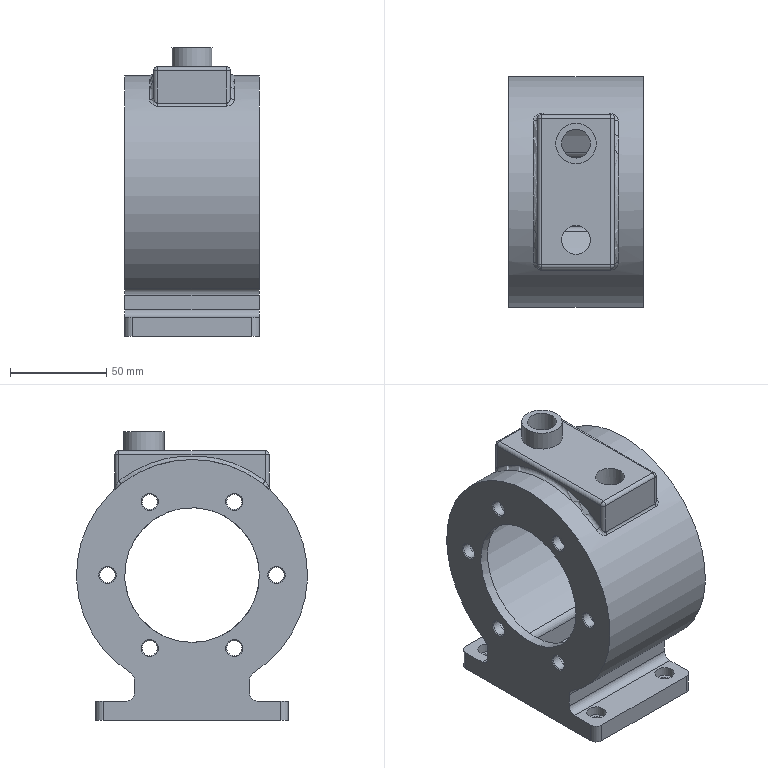Component | NX | HOUSING | 1 solid | 92 faces | volume 282967 mm3 | cylinder 46 | plane 24 | cone 12 | spline 4 | sphere 4 | torus 2 | commonest cylinder face diameters 8 x22 4 x9 6.6 x4 10 x4 70 x2 15 x2 110 x1 120 x1